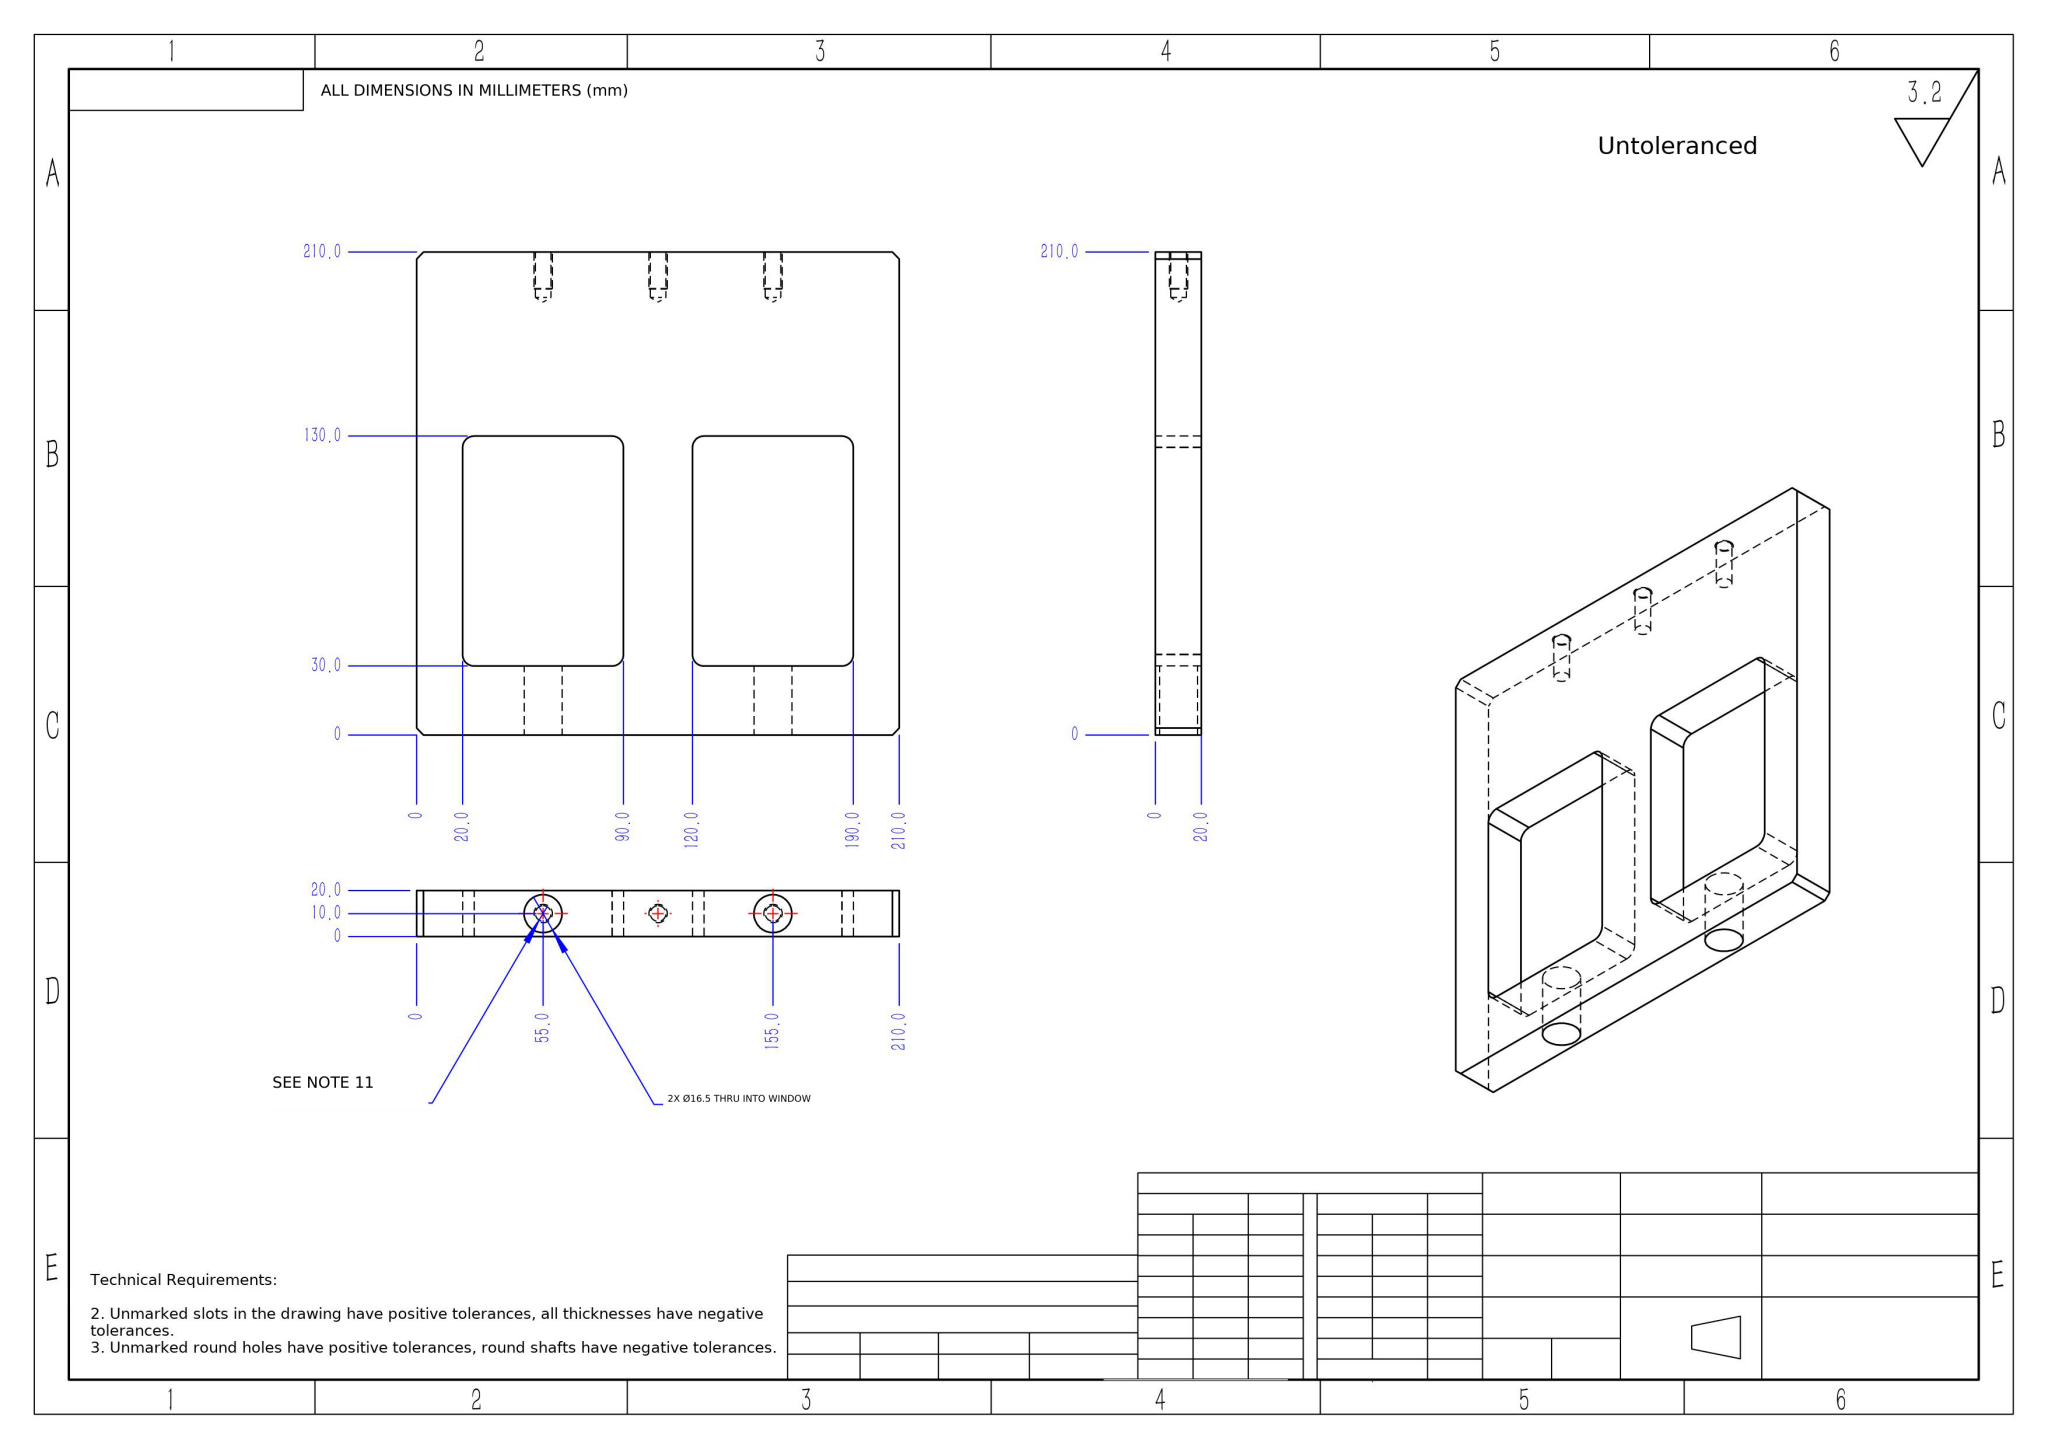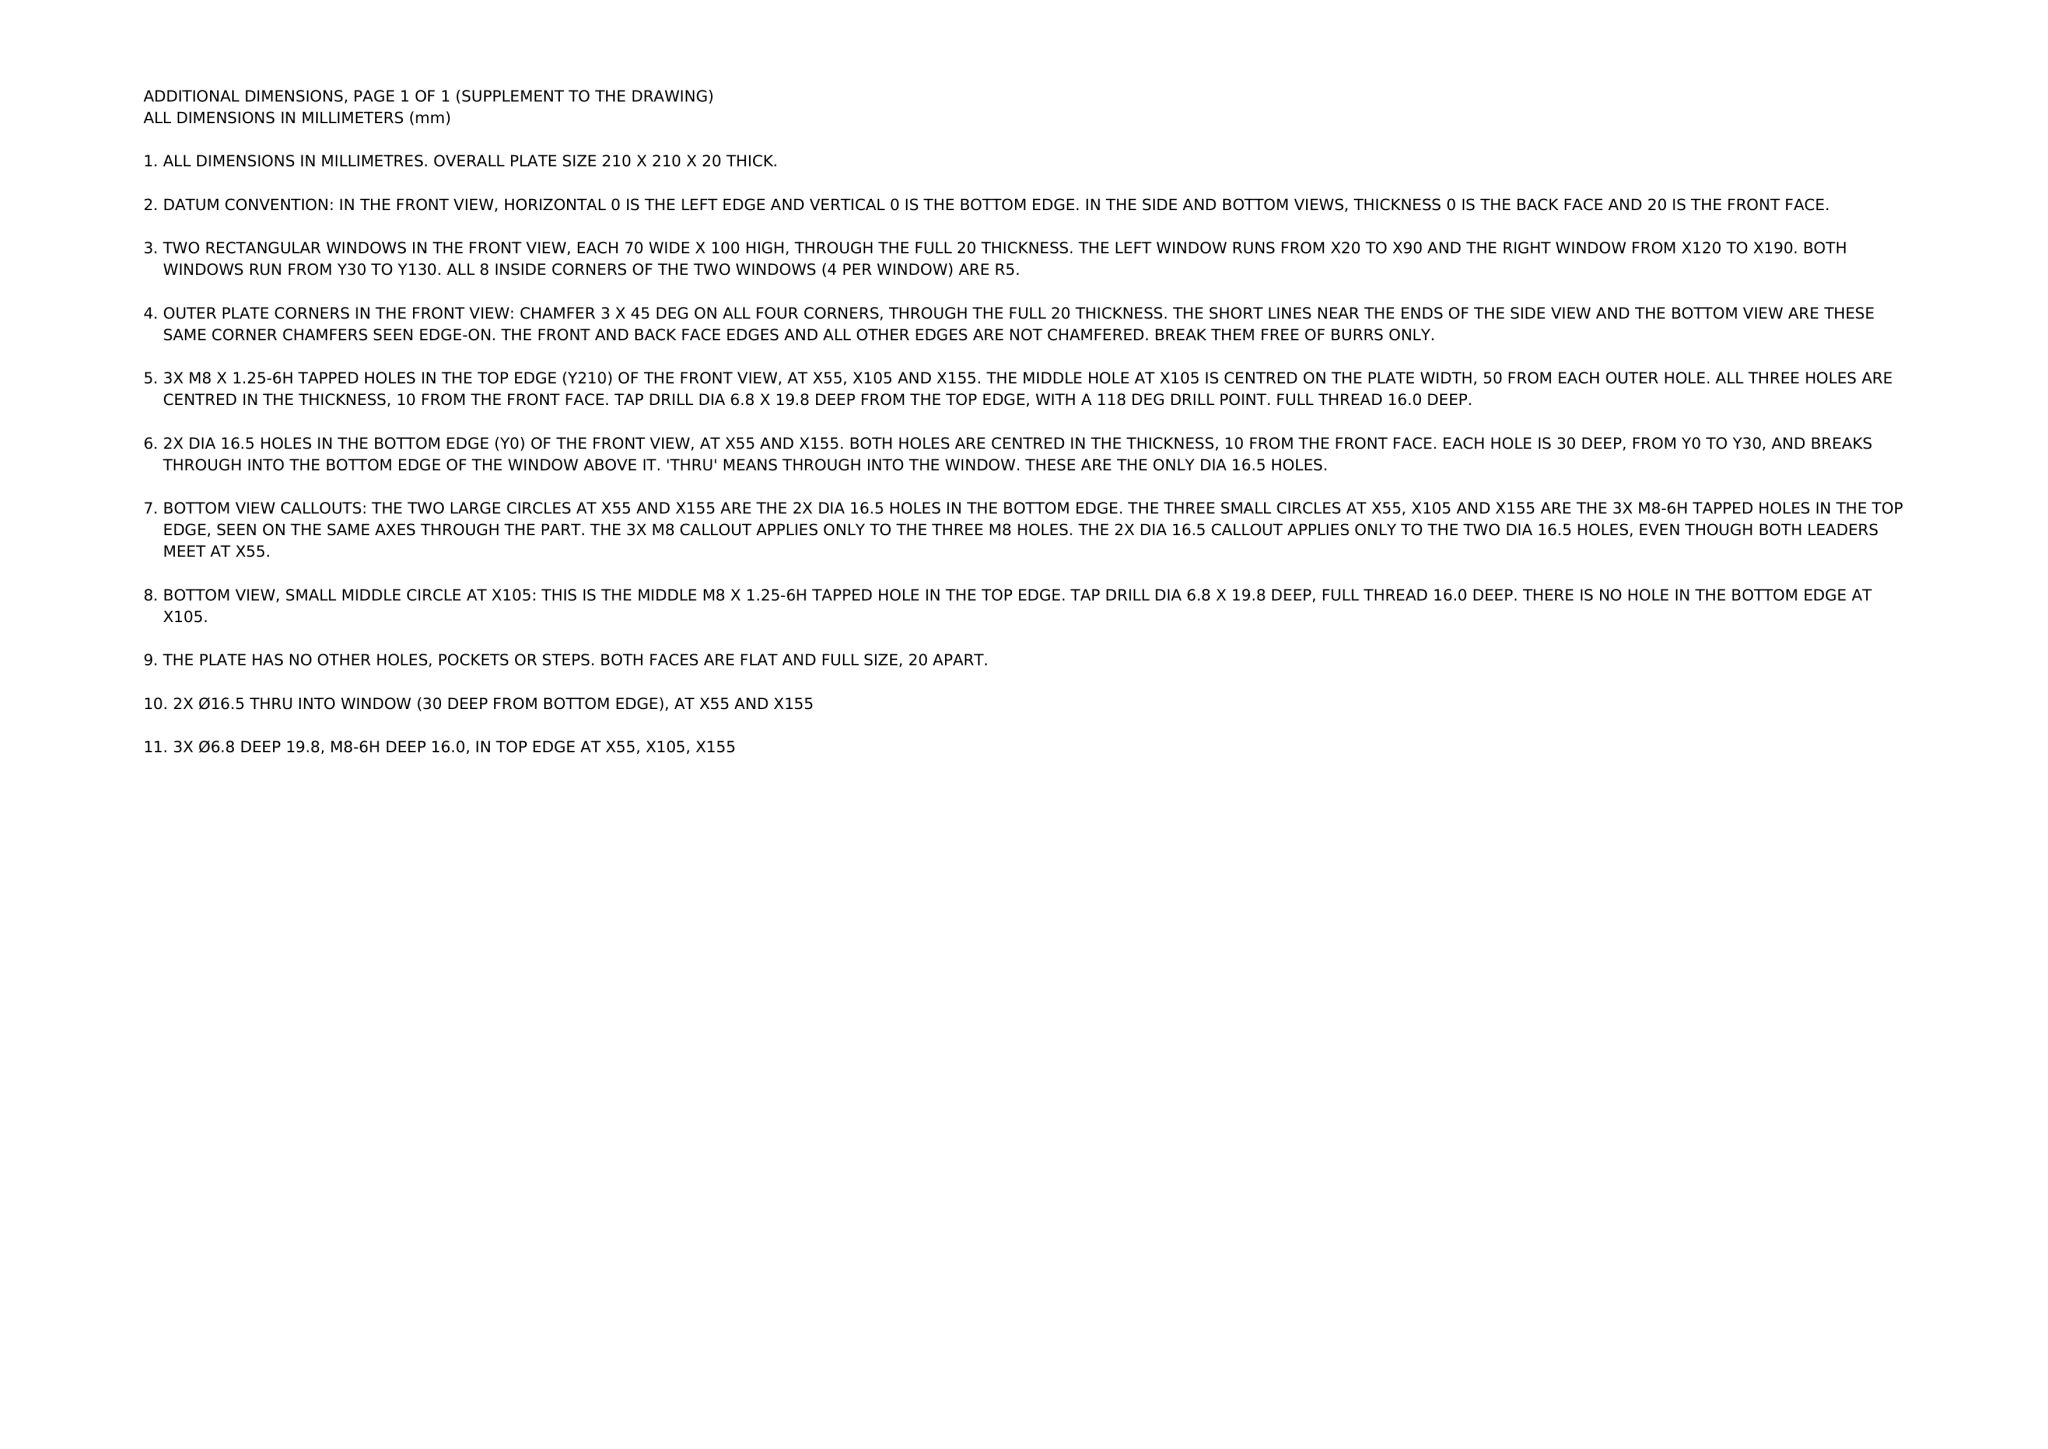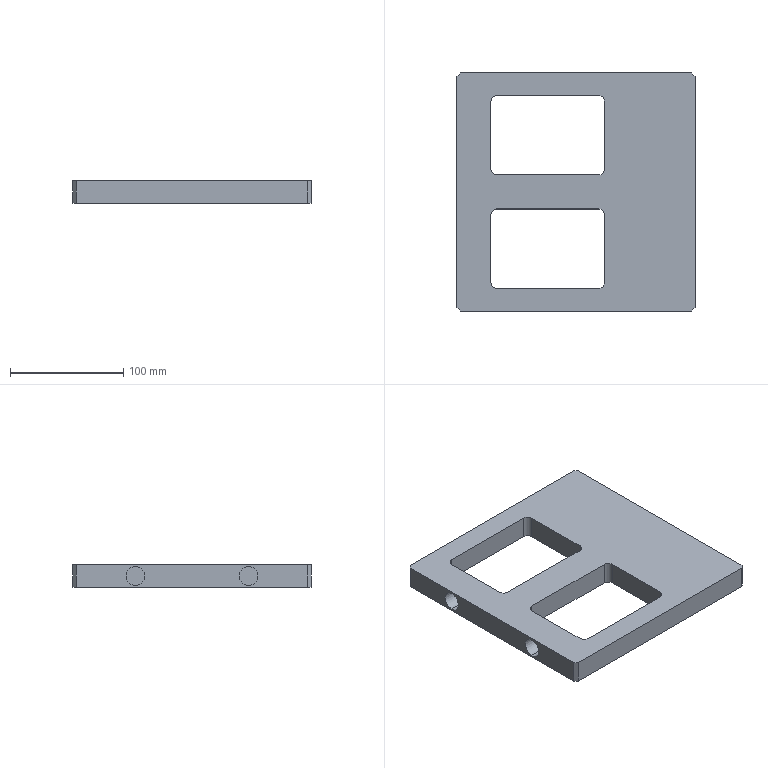Part | NX | mm | 1 solid | 42 faces | box 210 x 210 x 20 mm | volume 587443 mm3 | cylinder 18 | plane 18 | cone 6 | commonest cylinder face diameters 10 x8 6.8 x6 16.5 x4